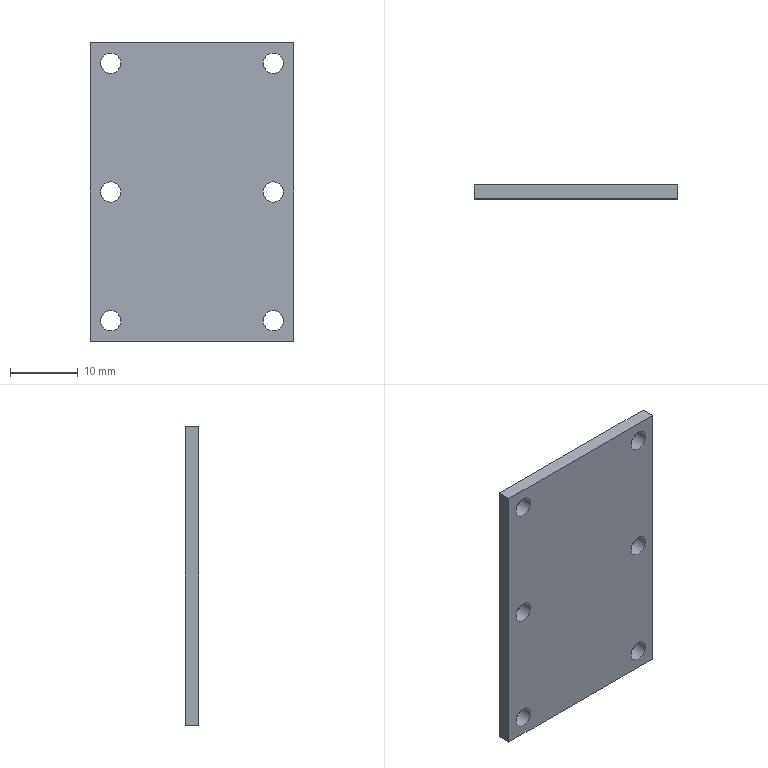Component | NX | WATER_CYL_TANK_END_PLATE | 1 solid | 12 faces | volume 2555 mm3 | plane 6 | cylinder 6 | commonest cylinder face diameters 3 x6